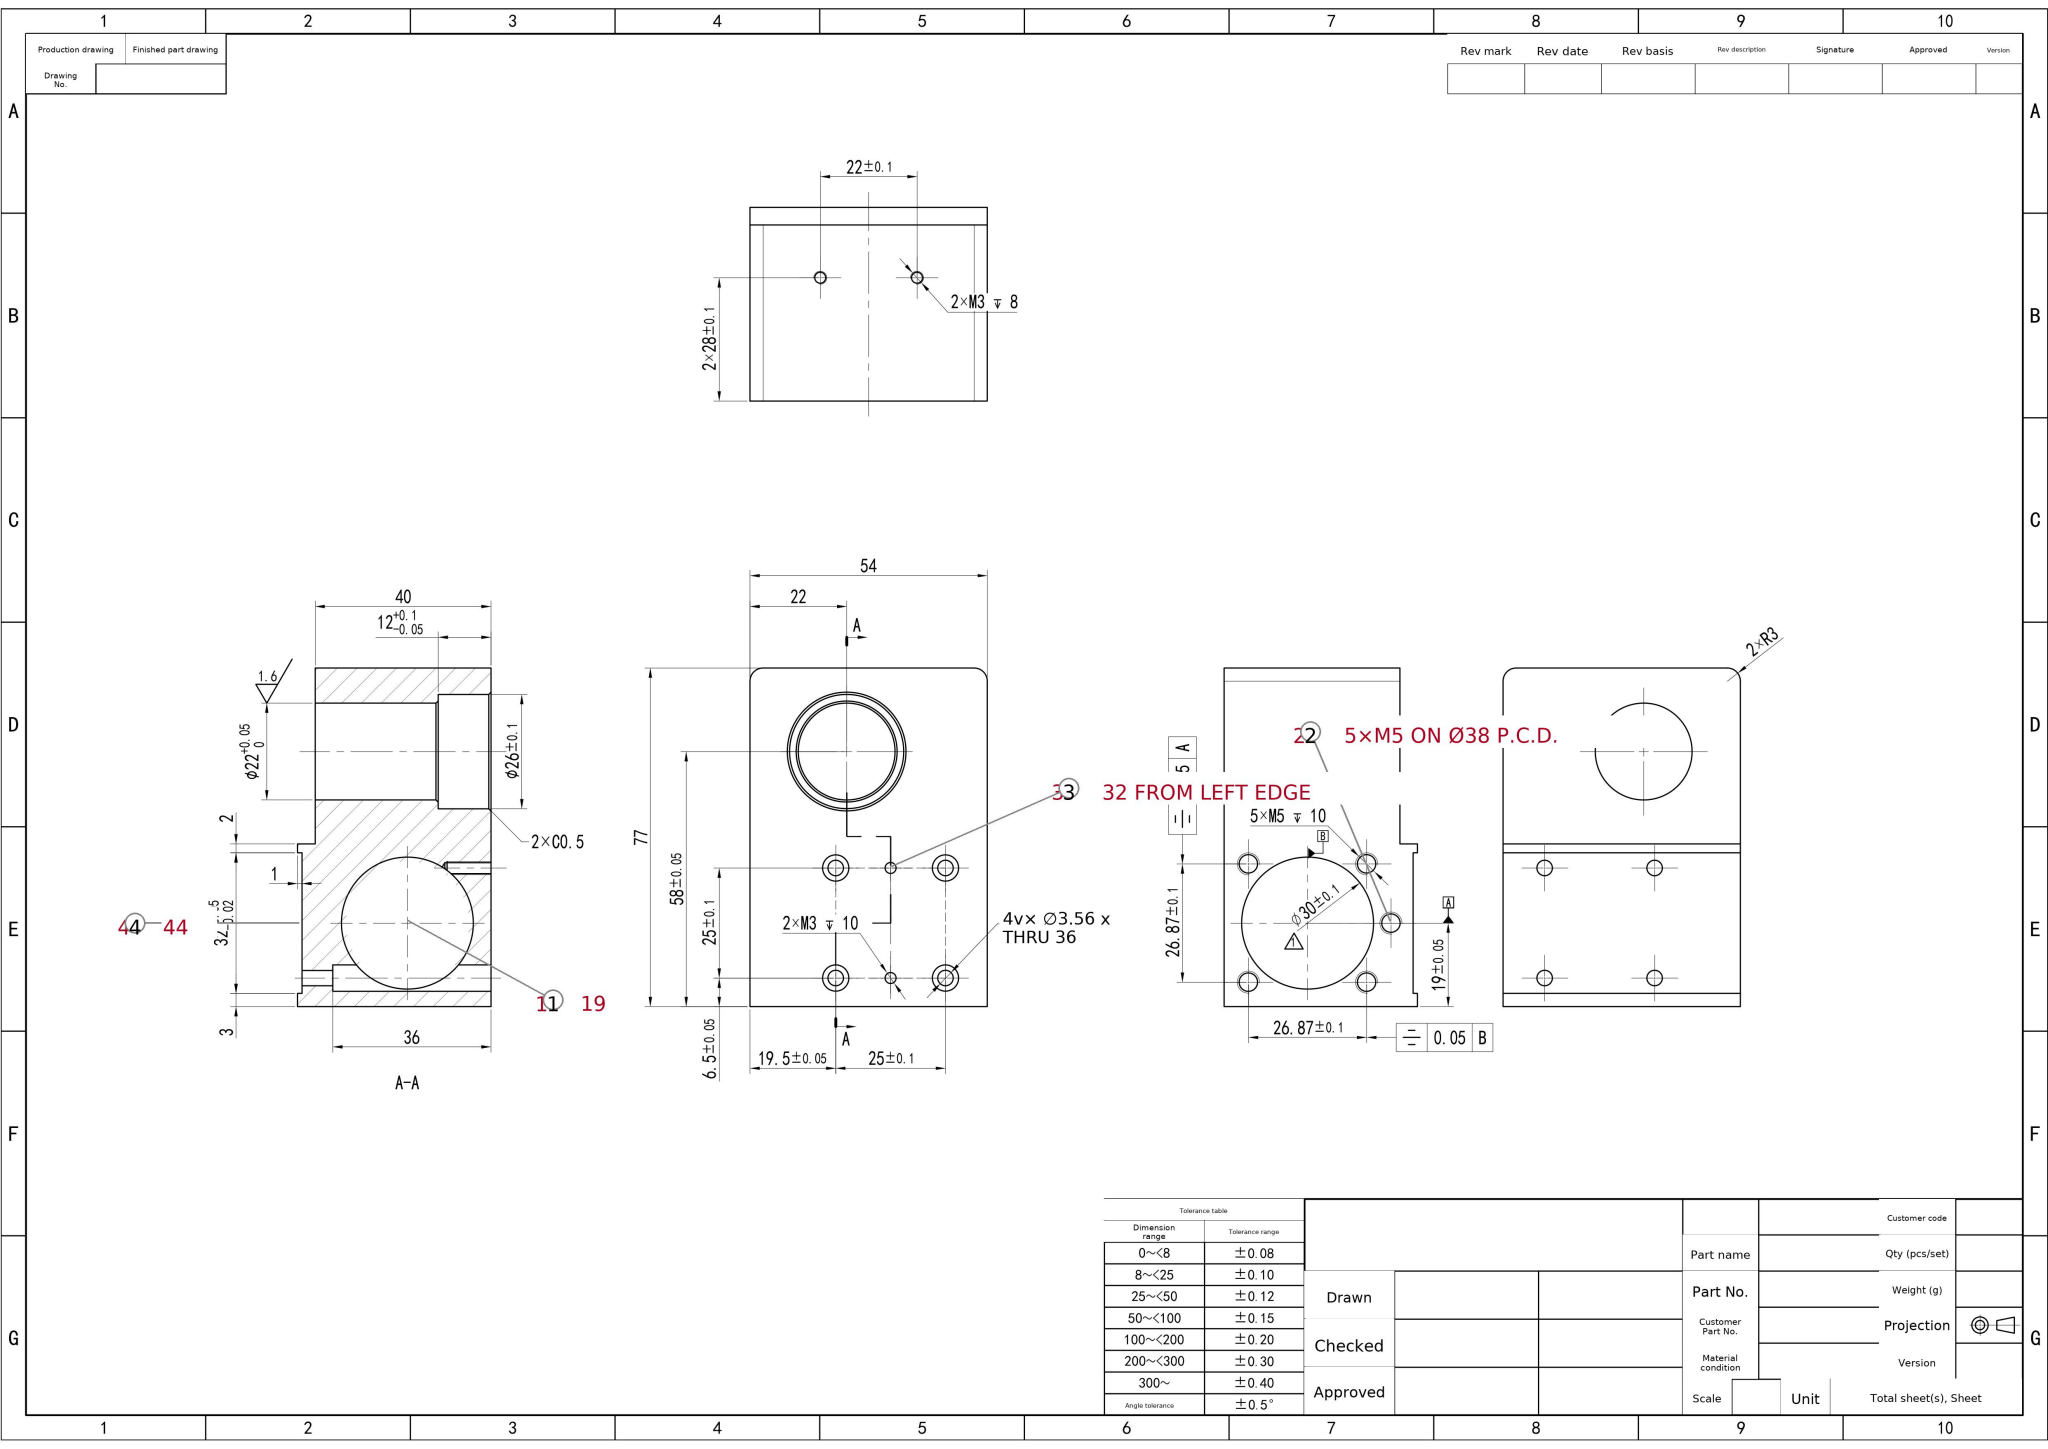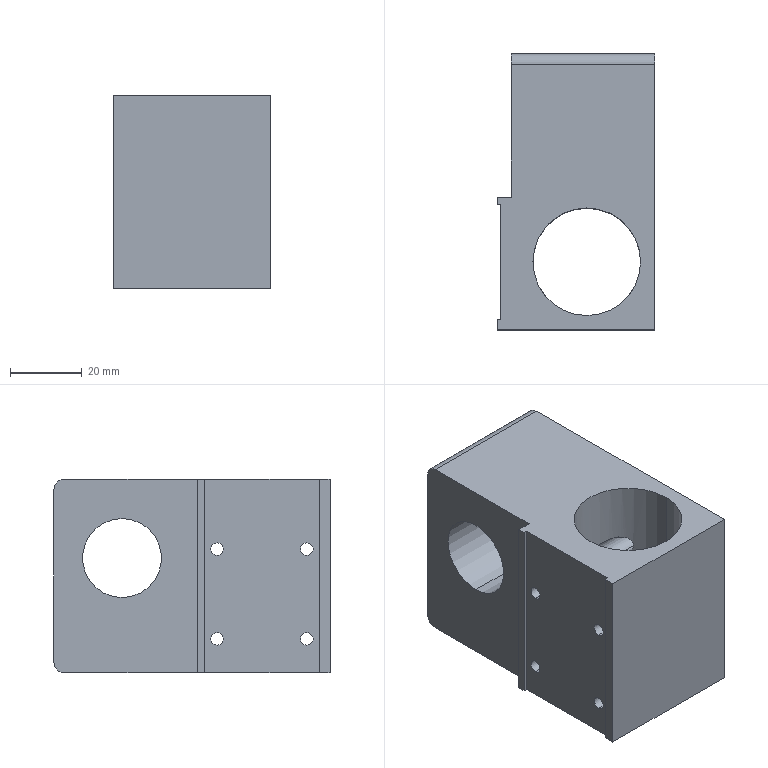Part | SolidWorks | mm | 1 solid | 82 faces | box 44 x 77 x 54 mm | volume 113915 mm3 | cylinder 46 | plane 22 | cone 14 | commonest cylinder face diameters 6 x14 4.2 x10 2.5 x8 3.5 x8 30 x2 22 x2 26 x2